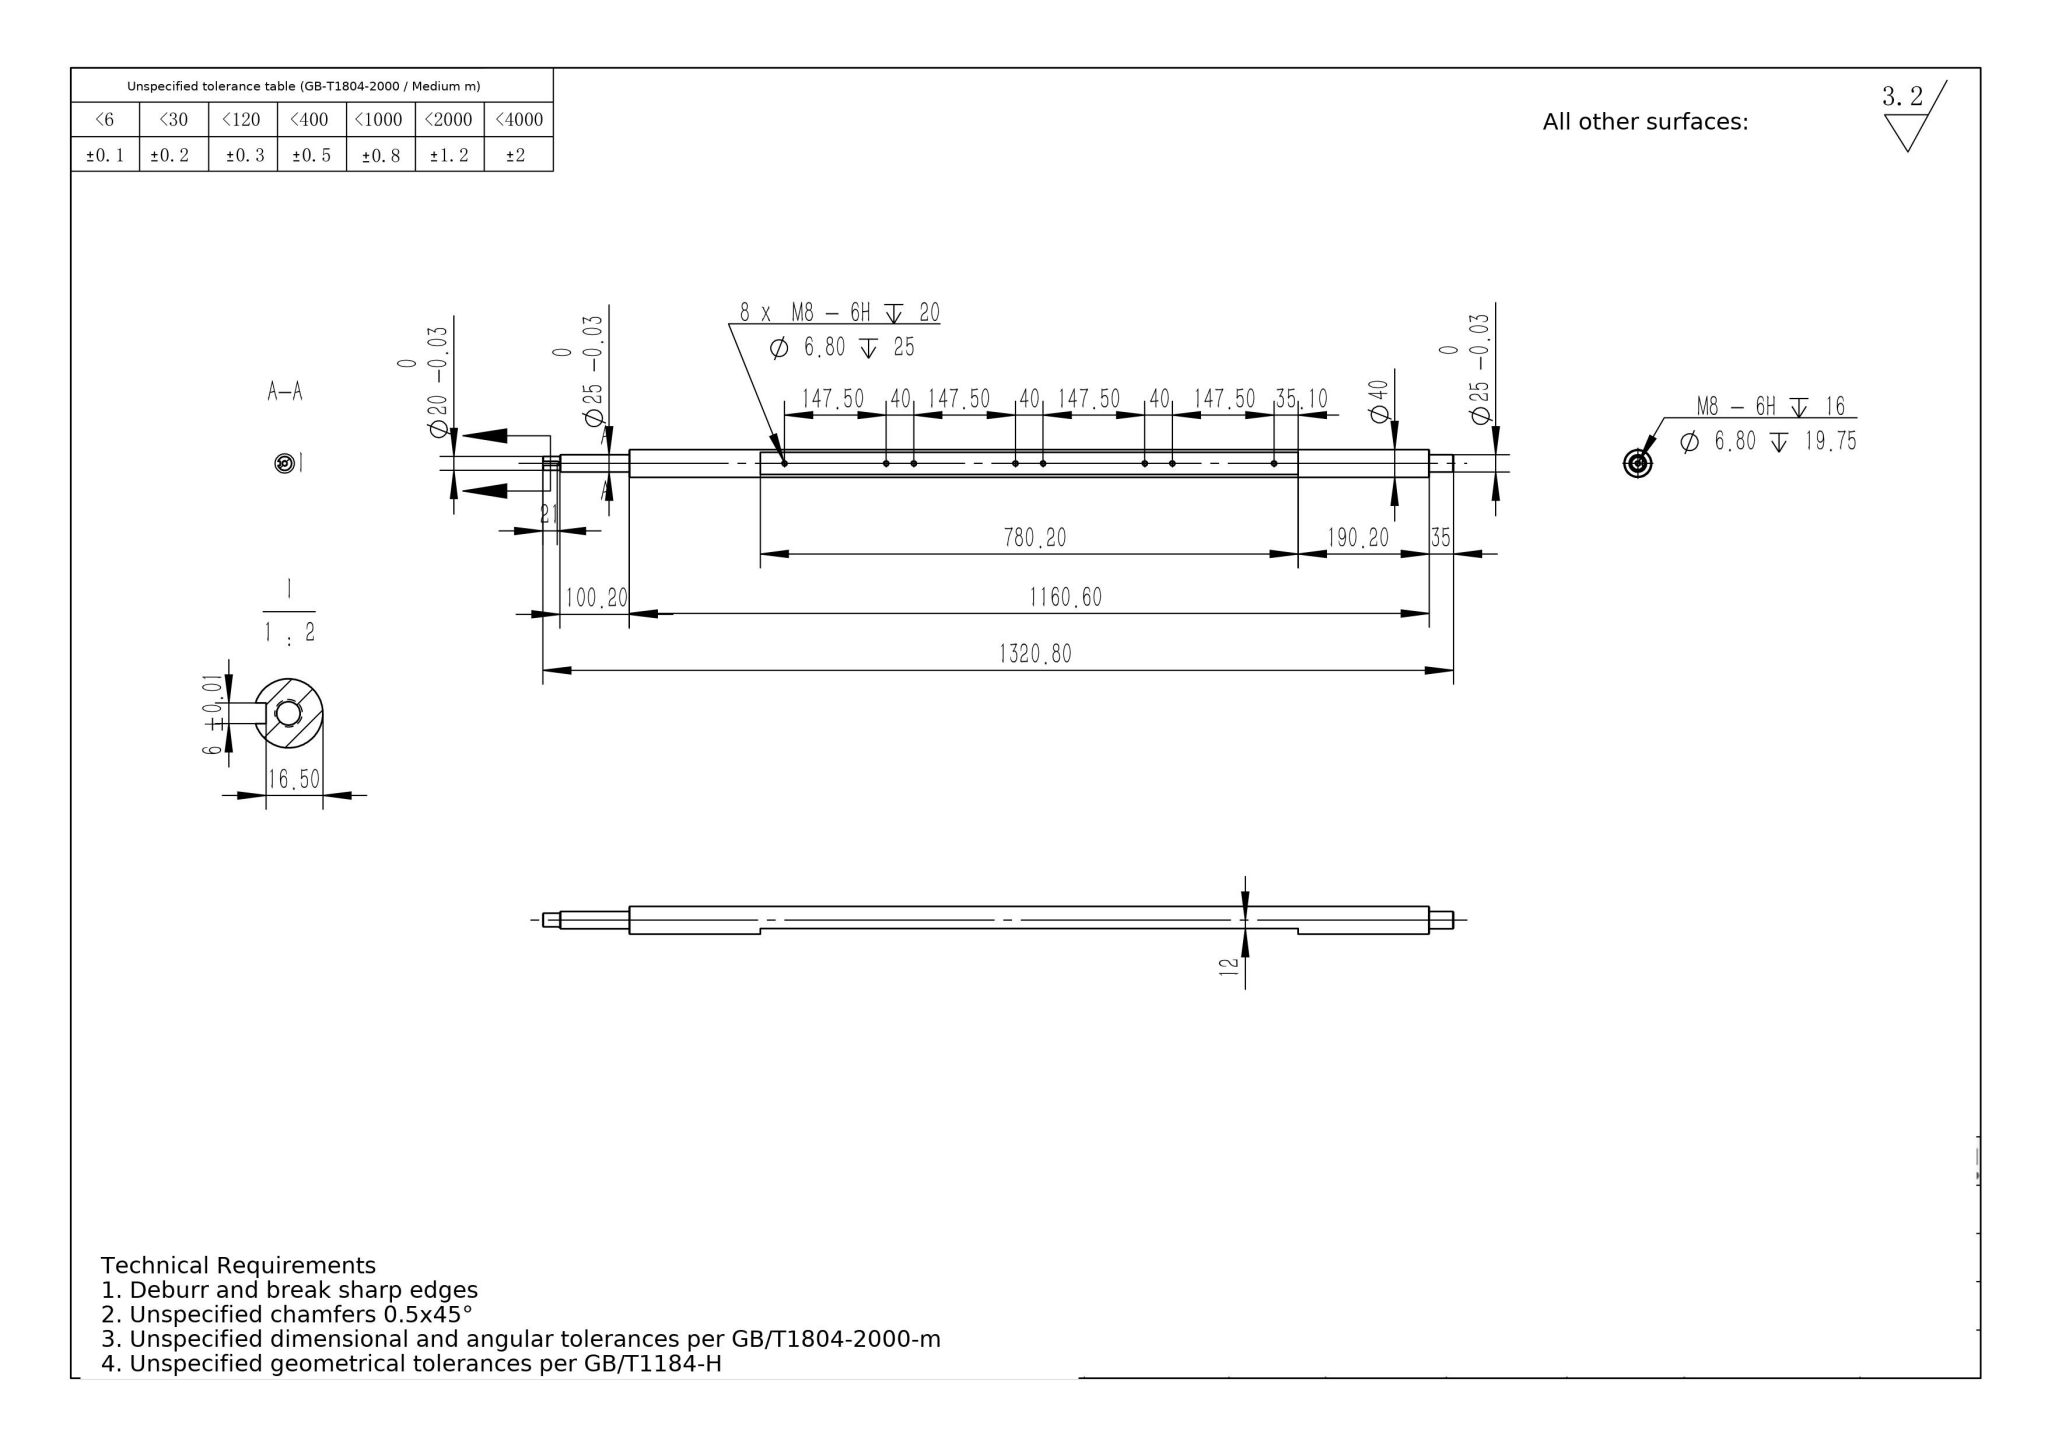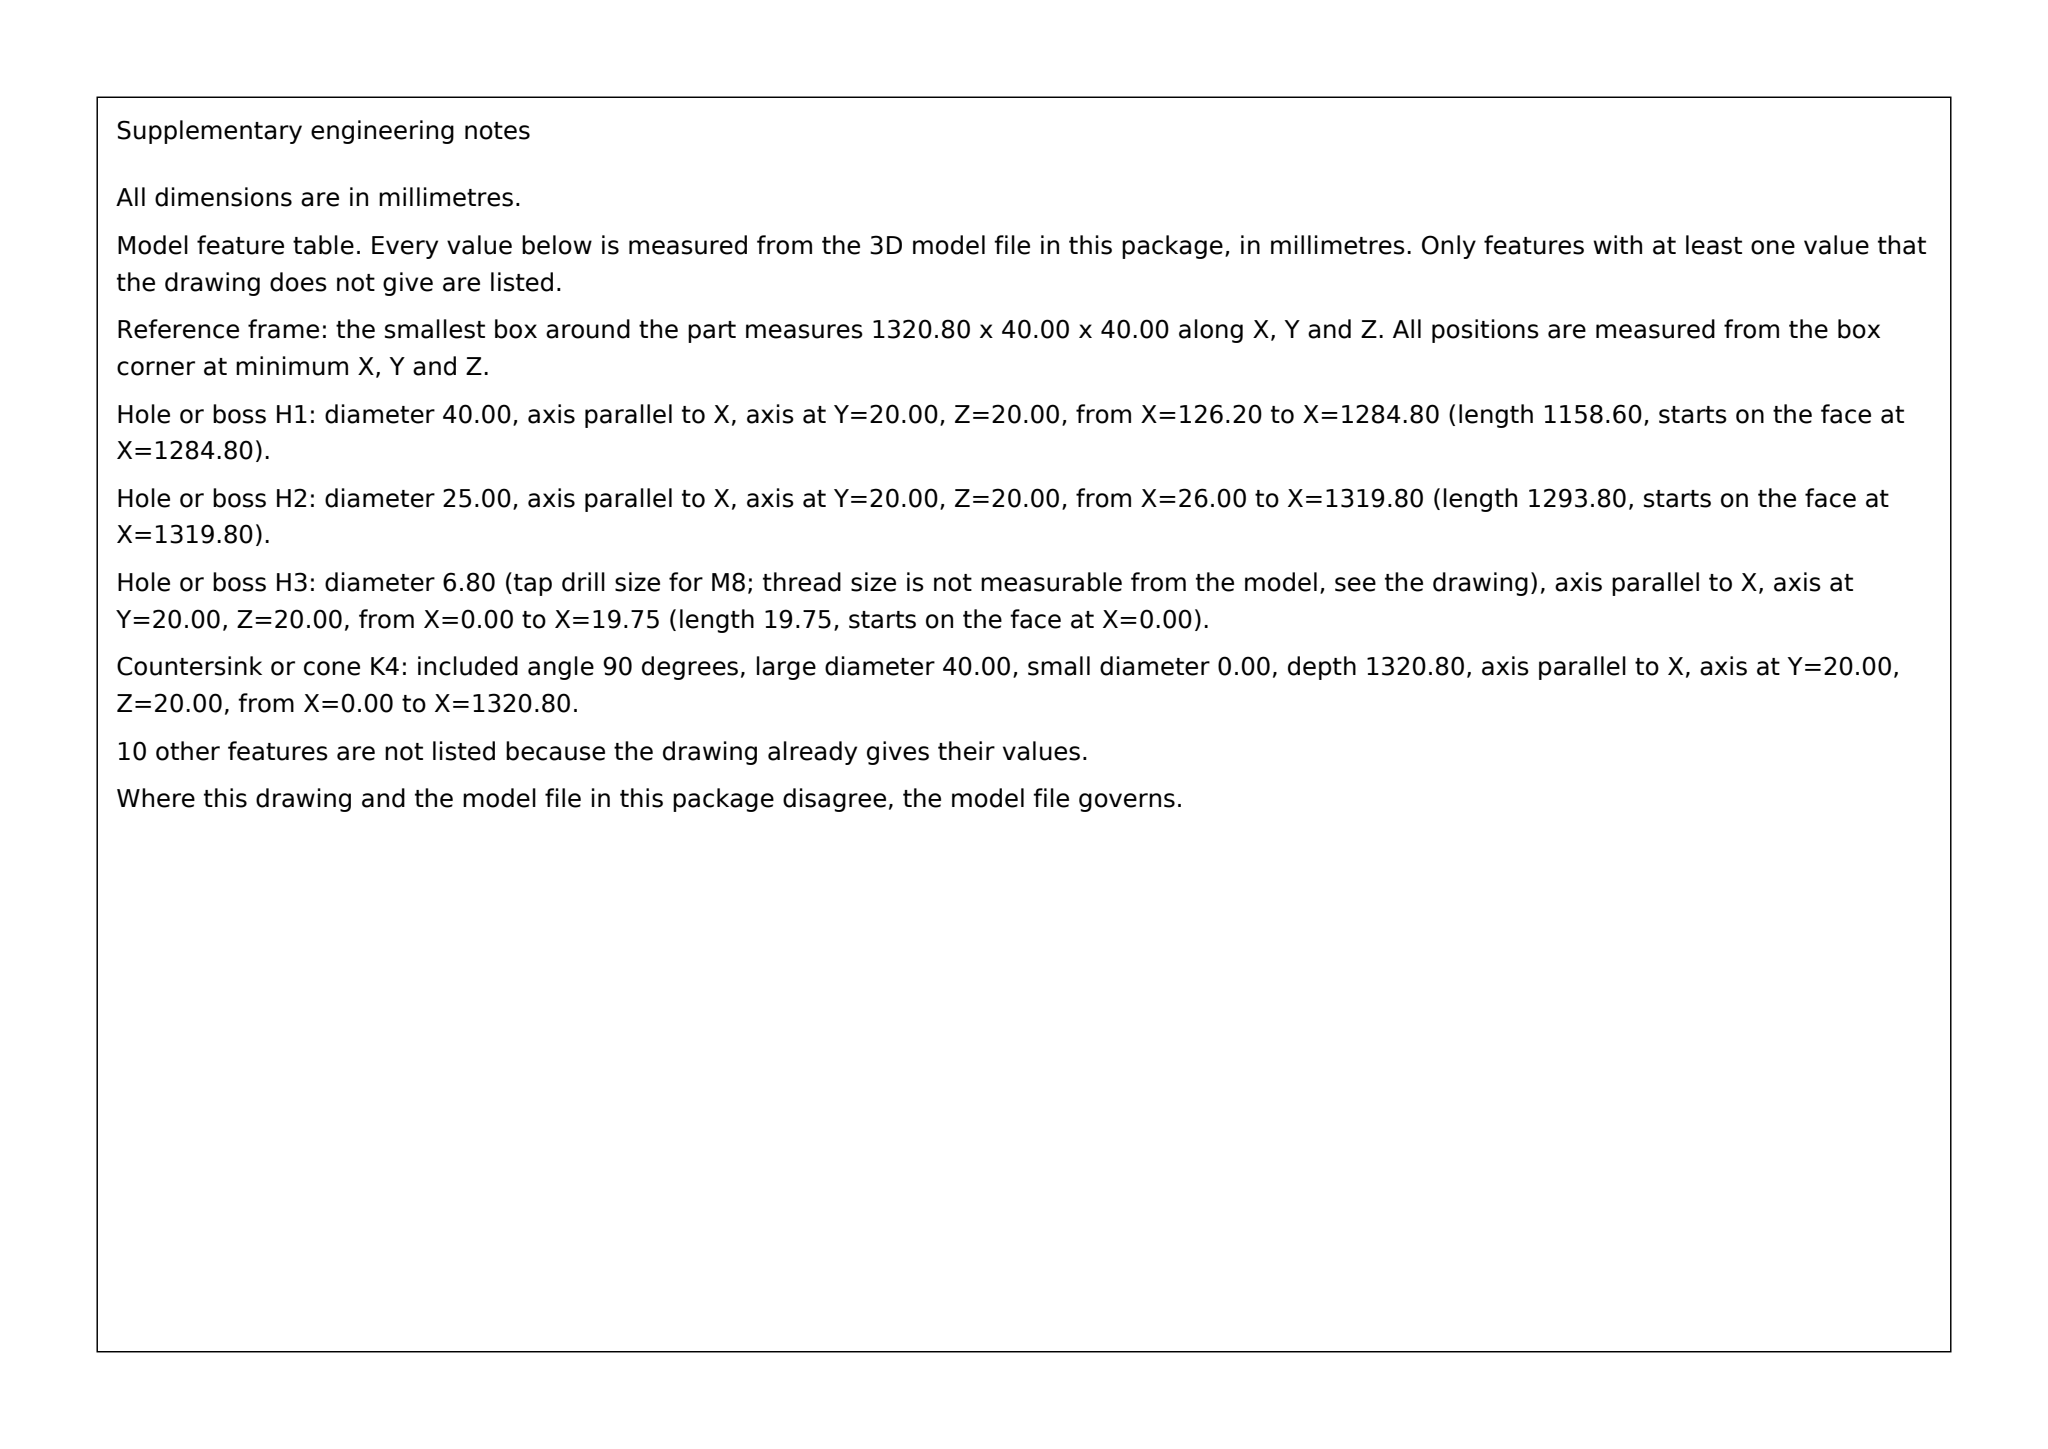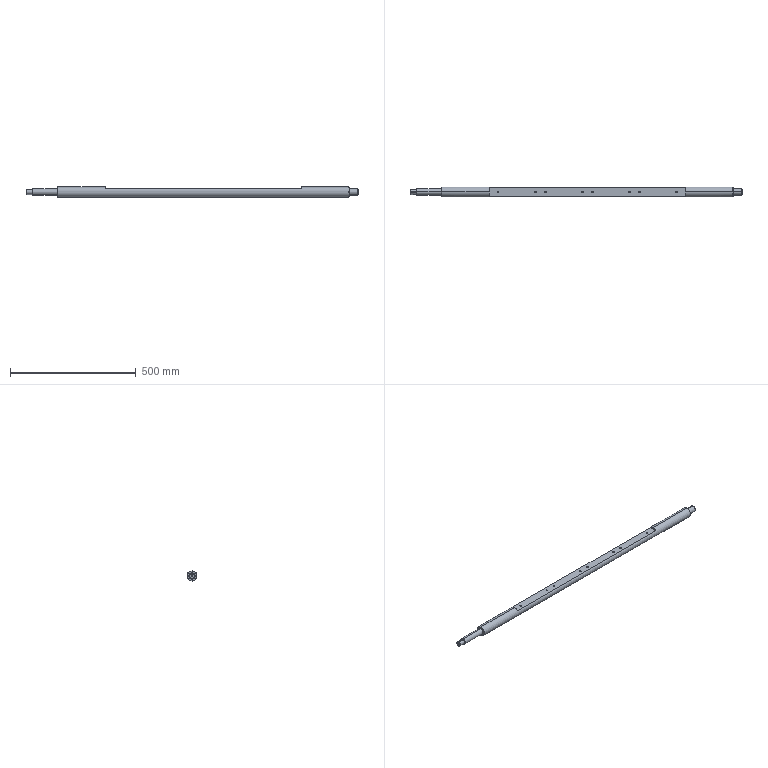Part | SolidWorks | mm | 1 solid | 67 faces | box 1320.8 x 40 x 40 mm | volume 1384181 mm3 | cone 28 | cylinder 28 | plane 11 | commonest cylinder face diameters 6.8 x18 25 x4 6 x2 20 x2 40 x2
build123d program:
from build123d import *

# Parameters (mm, degrees)
CUT_EXTRUDE1_START    = 10
CUT_EXTRUDE1_DEPTH    = 3.5
CUT_EXTRUDE2_START    = 20
SKETCH3_W             = 780.2
SKETCH3_H             = 40
CUT_EXTRUDE2_DEPTH    = 8
M8_TAPPED_HOLE1_D     = 6.8
M8_TAPPED_HOLE1_DEPTH = 25
M8_TAPPED_HOLE1_TIP   = 2.043
M8_TAPPED_HOLE2_D     = 6.8
M8_TAPPED_HOLE2_DEPTH = 19.75
M8_TAPPED_HOLE2_TIP   = 2.043
CHAMFER1_SIZE         = 1


with BuildPart() as part:
    # Sketch1 → Revolve1 (revolve)
    with BuildSketch(Plane.XY, mode=Mode.PRIVATE) as revolve1_sk:
        Polygon((25, 12.5), (25, 10), (0, 10), (0, 0), (1320.8, 0), (1320.8, 12.5), (1285.8, 12.5), (1285.8, 20), (125.2, 20), (125.2, 12.5), align=None)
    revolve(revolve1_sk.sketch.rotate(Axis((0, 0, 0), (-1, 0, 0)), 90), axis=Axis((0, 0, 0), (-1, 0, 0)))

    # Sketch2 → Cut-Extrude1 (cut)
    with BuildSketch(Plane.XY.offset(CUT_EXTRUDE1_START)):
        with BuildLine():
            Line((0, 3), (21, 3))
            ThreePointArc((21, 3), (24, 0), (21, -3))
            Line((21, -3), (0, -3))
            ThreePointArc((0, -3), (-3, 0), (0, 3))
        make_face()
    extrude(amount=-CUT_EXTRUDE1_DEPTH, mode=Mode.SUBTRACT)

    # Sketch3 → Cut-Extrude2 (cut)
    with BuildSketch(Plane.XY.offset(CUT_EXTRUDE2_START)):
        with Locations((705.5, 0)):
            Rectangle(SKETCH3_W, SKETCH3_H)
    extrude(amount=-CUT_EXTRUDE2_DEPTH, mode=Mode.SUBTRACT)

    # M8 Tapped Hole1
    with Locations(Plane.XY.offset(12)):
        with Locations((350.5, 0), (498, 0), (538, 0), (685.5, 0), (725.5, 0), (873, 0), (913, 0), (1060.5, 0)):
            Hole(M8_TAPPED_HOLE1_D / 2, depth=M8_TAPPED_HOLE1_DEPTH)
            with Locations((0, 0, -(M8_TAPPED_HOLE1_DEPTH + M8_TAPPED_HOLE1_TIP / 2))):  # 118° drill point
                Cone(0, M8_TAPPED_HOLE1_D / 2, M8_TAPPED_HOLE1_TIP, mode=Mode.SUBTRACT)

    # M8 Tapped Hole2
    with Locations(Plane.ZY):
        with Locations((0, 0)):
            Hole(M8_TAPPED_HOLE2_D / 2, depth=M8_TAPPED_HOLE2_DEPTH)
            with Locations((0, 0, -(M8_TAPPED_HOLE2_DEPTH + M8_TAPPED_HOLE2_TIP / 2))):  # 118° drill point
                Cone(0, M8_TAPPED_HOLE2_D / 2, M8_TAPPED_HOLE2_TIP, mode=Mode.SUBTRACT)

    # Chamfer1
    chamfer1_edges = [part.edges().sort_by_distance(p)[0] for p in [
        (25, 0, 12.5),
        (0, 9.884, -1.518),
        (1320.8, 0, 12.5),
        (1285.8, 0, 20),
        (125.2, 0, 20),
    ]]
    chamfer(chamfer1_edges, length=CHAMFER1_SIZE)


solid = part.part